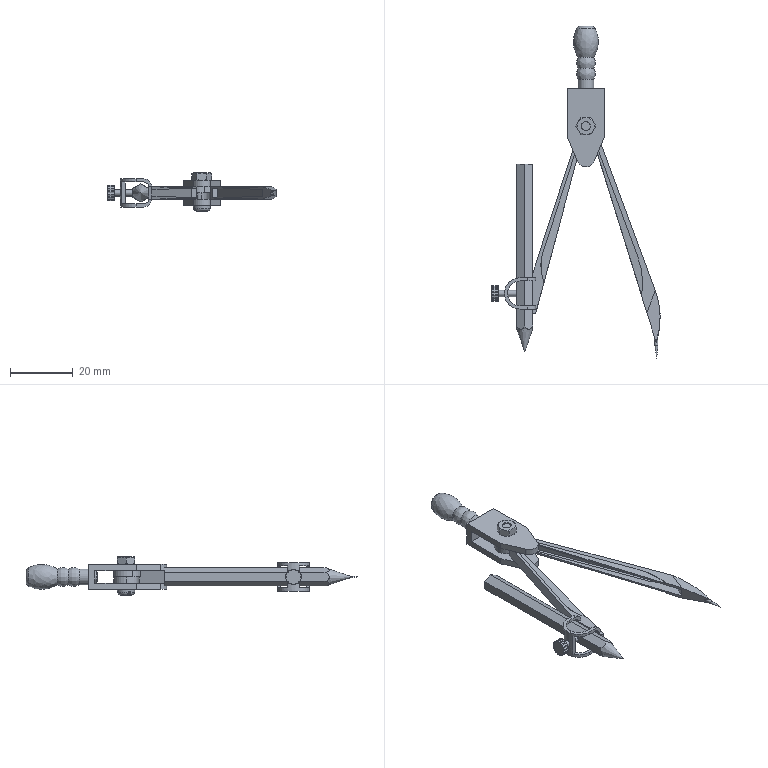Assembly | NX | mm | 9 component files | 9 solids | 200 faces | box 53.79 x 106.15 x 12.2 mm | volume 4071 mm3 | plane 101 | cylinder 72 | cone 20 | torus 4 | spline 3 | commonest cylinder face diameters 5 x21 0.9 x16 6 x6 8 x5 3.1 x4 3 x4 50 x3 4 x2
Bill of materials:
unnamed part 1 | 1 |  | U-shaped forked block: two parallel flat prongs joined by a solid back web, with tapered sides that narrow to rounded tips, and one round hole passing through both prongs.
unnamed part 2 | 1 |  | Straight rod with a hexagonal cross-section and a faceted conical point at one end; the other end is flat.
unnamed part 3 | 1 |  | Round turned part that looks like a handle: a two-step cylindrical spigot with a chamfered end, then two rounded bead rings, then a large barrel-shaped bulb at the other end.
unnamed part 4 | 1 |  | Hexagonal prism with a central round through-bore and chamfered (curved-edge) corners on both faces, like a hex nut.
unnamed part 5 | 1 |  | Long thin flat strip with a round eyelet (ring with a hole) at one end; the other end tapers to a slightly curved point with a small notch at the tip.
unnamed part 6 | 1 |  | Plain cylindrical rod with a long conical taper to a sharp point at one end and a flat other end.
unnamed part 7 | 1 |  | Pin with a scalloped (fluted) round head and a plain cylindrical shank with a chamfered free end.
unnamed part 8 | 1 |  | Long flat tapered arm with a round eyelet at one end and a thin-walled D-shaped open loop or band frame at the other end, set crosswise to the arm.
unnamed part 9 | 1 |  | Headed pin: a cylindrical shank on a wider round head with a rounded underside edge. There is a short neck or groove where the shank meets the head, and a small notch in the side of the head.
Mates:
1. fix | 01 1 component
2. concentric | 01 1 edge | 02 1 arc
3. concentric | 03 1 edge | 02 1 edge
4. touch align | 03 1 face | 02 1 face
5. concentric | 04 1 edge | 03 1 edge
6. concentric | 05 1 edge | 03 1 edge
7. touch align | 06 1 face | 05 1 face
8. parallel | 03 1 face | assembly datumplane
9. parallel | 05 1 face | assembly datumplane
10. parallel | 06 1 face | assembly datumplane
11. center | 06 1 edge | 06 1 edge | assembly datumplane
12. touch align | 07 1 face | 06 1 face
13. touch align | 07 1 face | 05 1 face